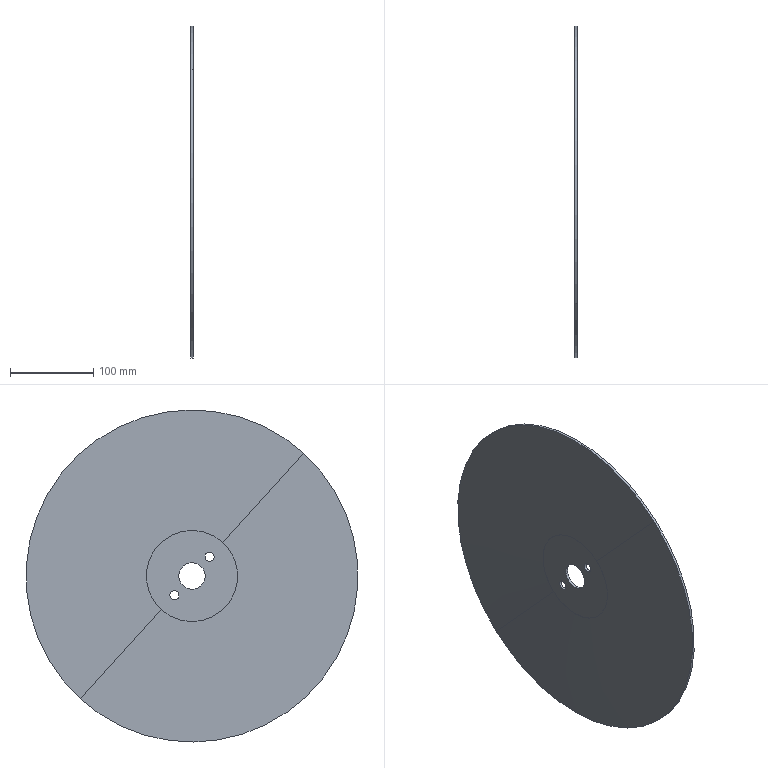Component | SolidWorks | SawBlade400-1 | 1 solid | 18 faces | box 3 x 400 x 400 mm | volume 355180 mm3 | cylinder 12 | cone 4 | plane 2 | commonest cylinder face diameters 110 x4 11 x4 32 x2 400 x2
build123d program:
from build123d import *

# Parameters (mm, degrees)
SKETCH1_R           = 200
SKETCH1_R_2         = 16
SKETCH1_R_3         = 5.5
BOSS_EXTRUDE1_DEPTH = 3


with BuildPart() as part:
    # Sketch1 → Boss-Extrude1 (new body)
    with BuildSketch(Plane.XY):
        Circle(SKETCH1_R)
        Circle(SKETCH1_R_2, mode=Mode.SUBTRACT)
        with Locations((-31.5, 0)):
            Circle(SKETCH1_R_3, mode=Mode.SUBTRACT)
        with Locations((31.5, 0)):
            Circle(SKETCH1_R_3, mode=Mode.SUBTRACT)
    extrude(amount=BOSS_EXTRUDE1_DEPTH)

    # Sketch3 → Cut-Revolve1 (revolve, cut)
    with BuildSketch(Plane(origin=(0, 0, 0), x_dir=(1, 0, 0), z_dir=(0, 1, 0)), mode=Mode.PRIVATE) as cut_revolve1_sk:
        Polygon((200, 0), (55, -0.2), (55, 0), align=None)
        Polygon((200, -3), (55, -2.8), (55, -3), align=None)
    revolve(cut_revolve1_sk.sketch.rotate(Axis((0, 0, 0), (0, 0, 1)), 180), axis=Axis((0, 0, 0), (0, 0, 1)), mode=Mode.SUBTRACT)


solid = part.part

# Placed as in the assembly
solid = solid.moved(Location((-159.809, -4.181, 0), (-137.789, 90, 0)))